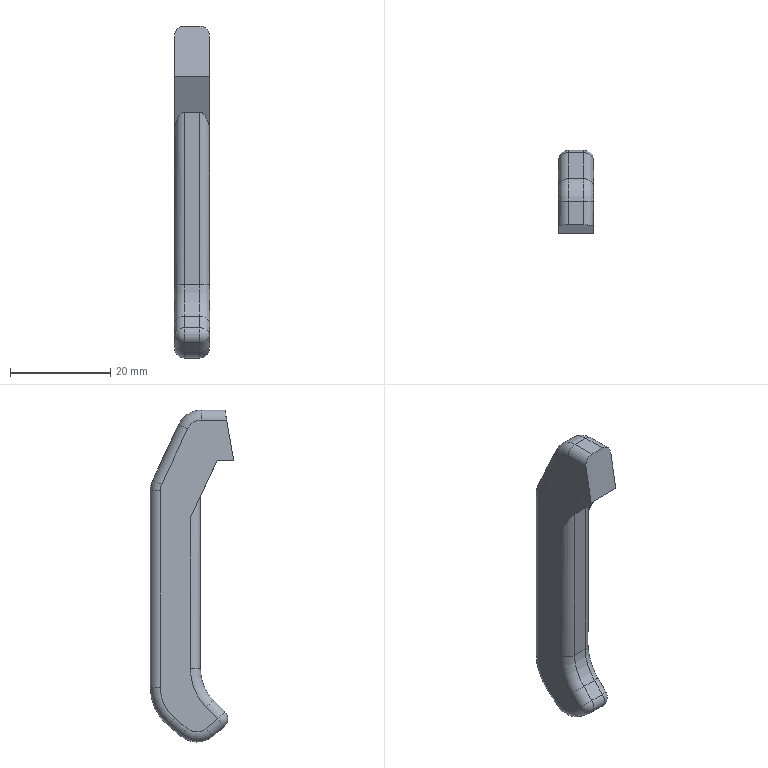Component | NX | MODEL28 | 1 solid | 44 faces | volume 4602 mm3 | cylinder 20 | plane 12 | torus 10 | sphere 2 | commonest cylinder face diameters 4 x15 10 x3 20 x1 17.901 x1